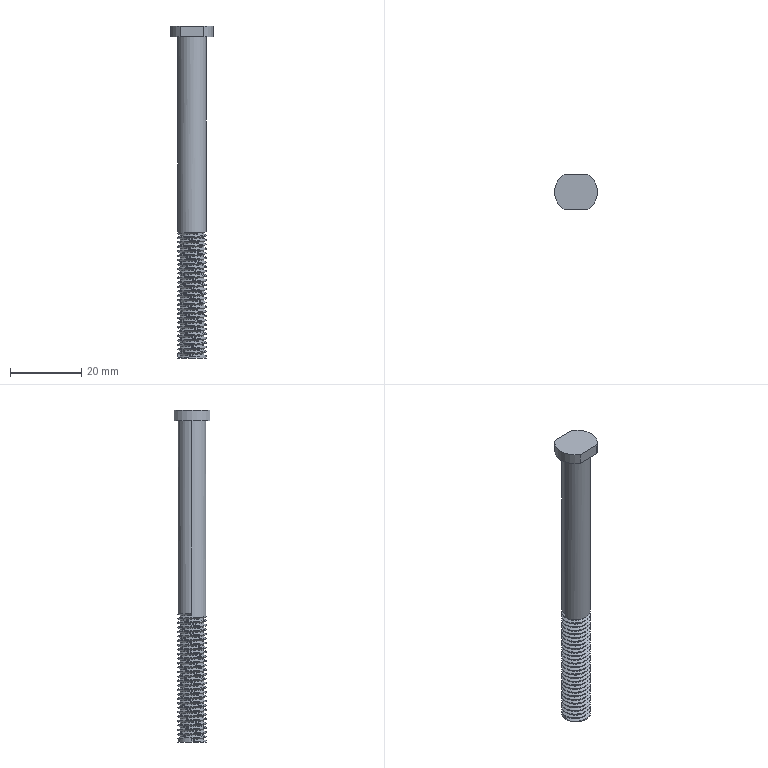Component | SolidWorks | GuideRod-2 | 1 solid | 71 faces | volume 4528 mm3 | cylinder 61 | plane 7 | spline 3 | commonest cylinder face diameters 8 x58 12 x3